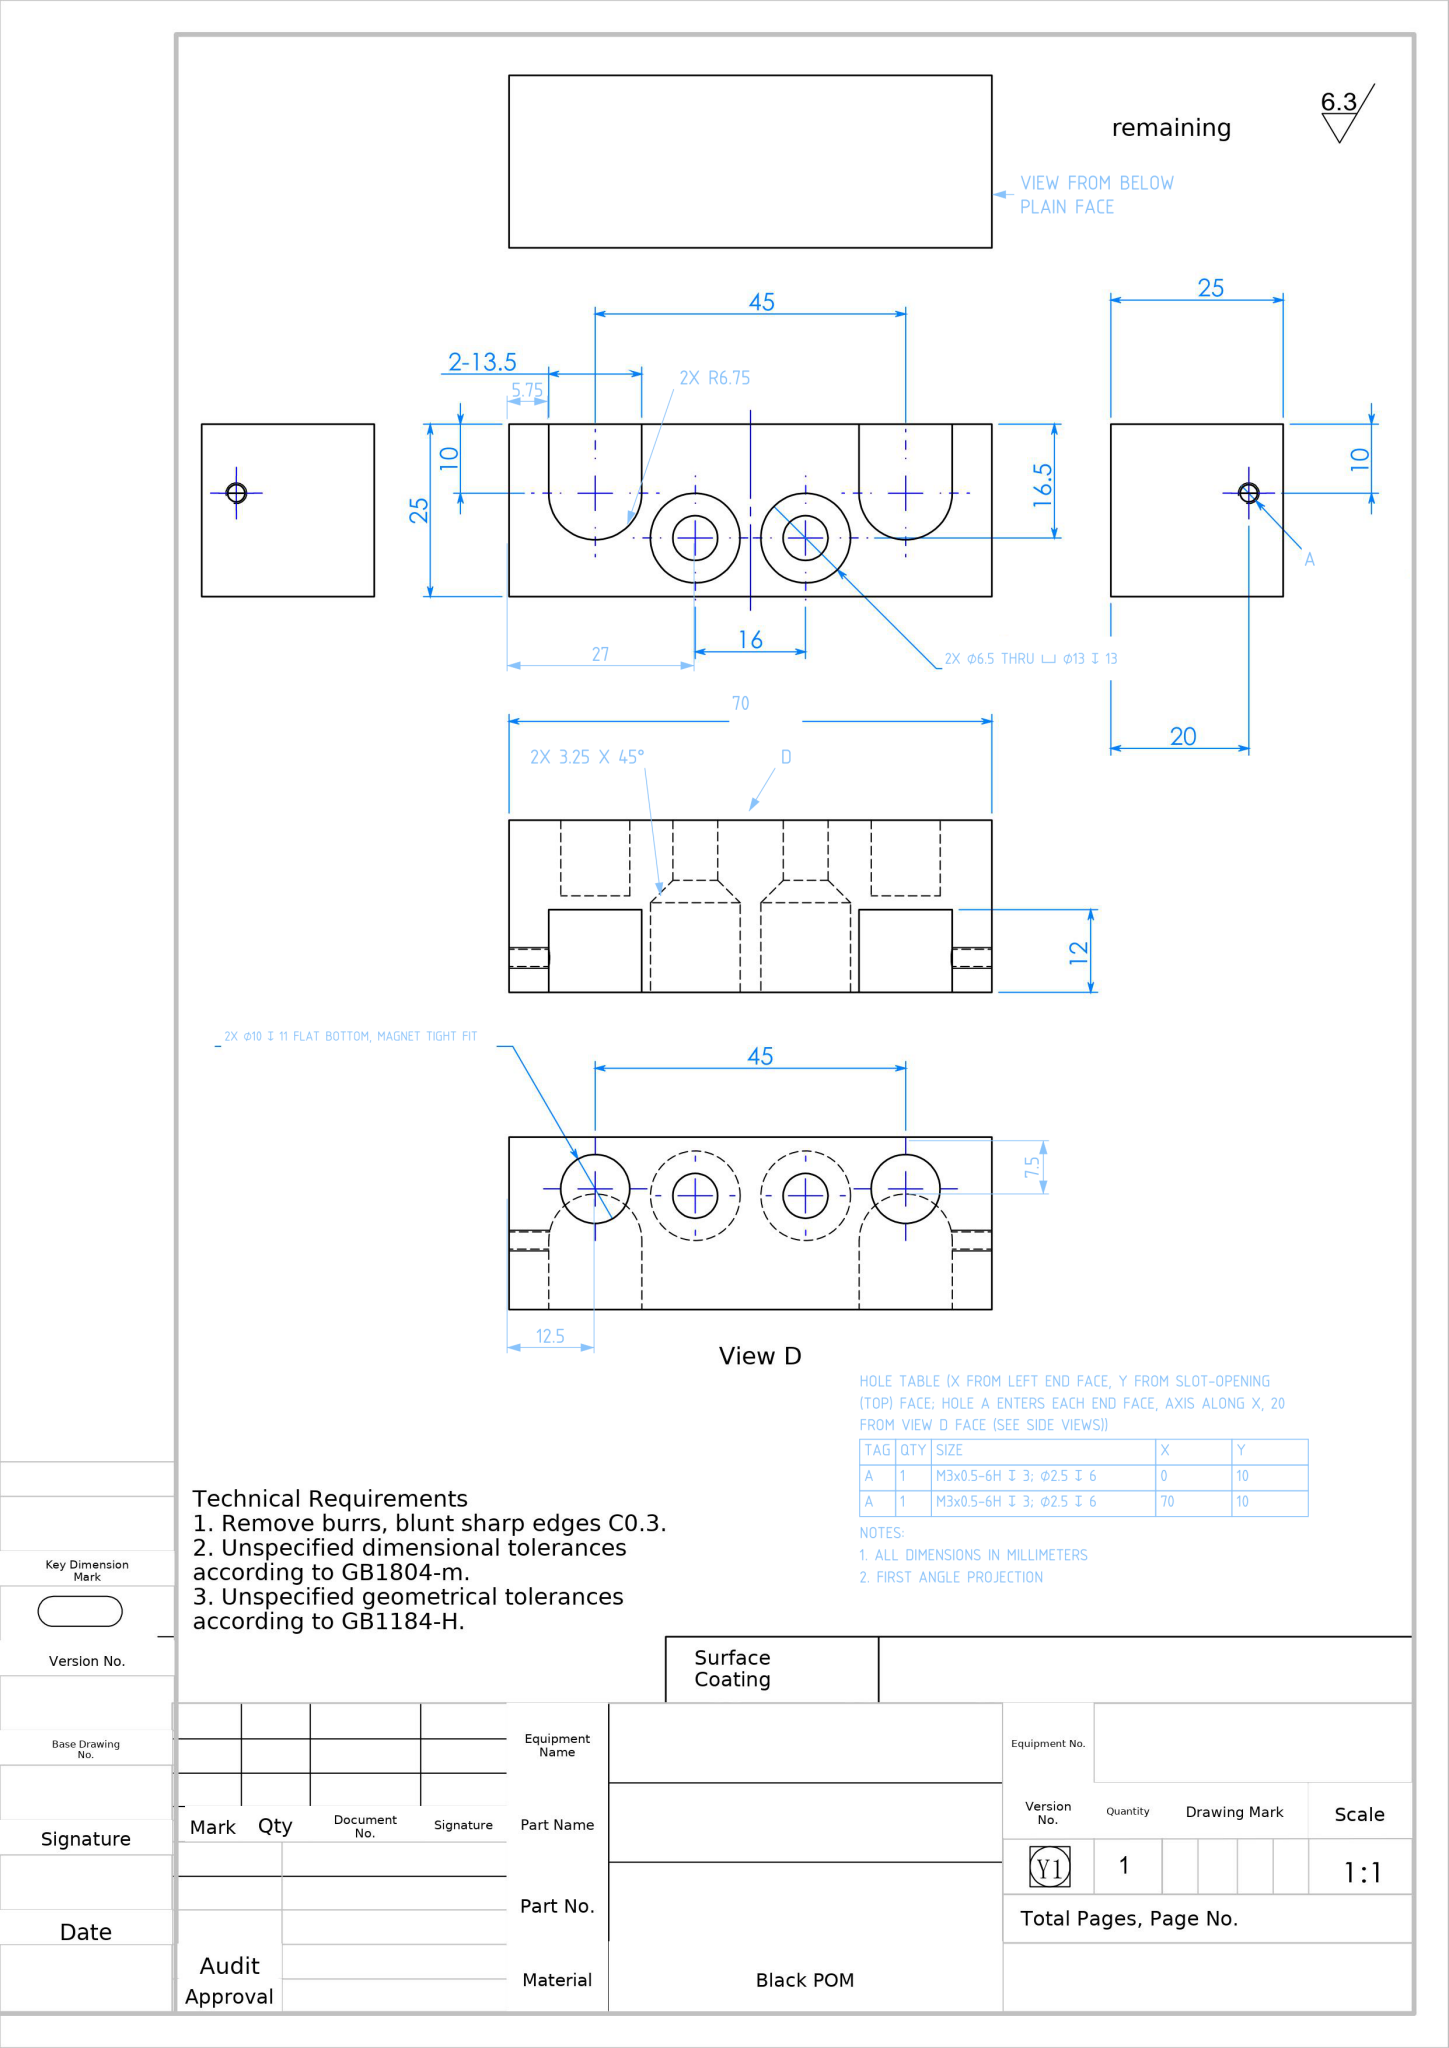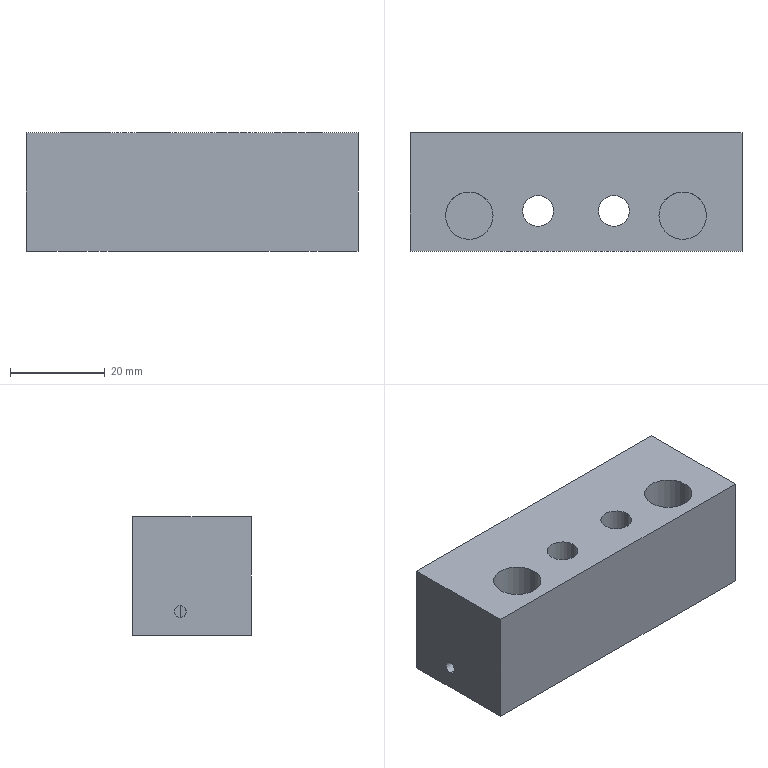Part | NX | mm | 1 solid | 36 faces | box 70 x 25 x 25 mm | volume 32473 mm3 | cylinder 18 | plane 14 | cone 4 | commonest cylinder face diameters 10 x4 2.5 x4 6.5 x4 13 x4 13.5 x2